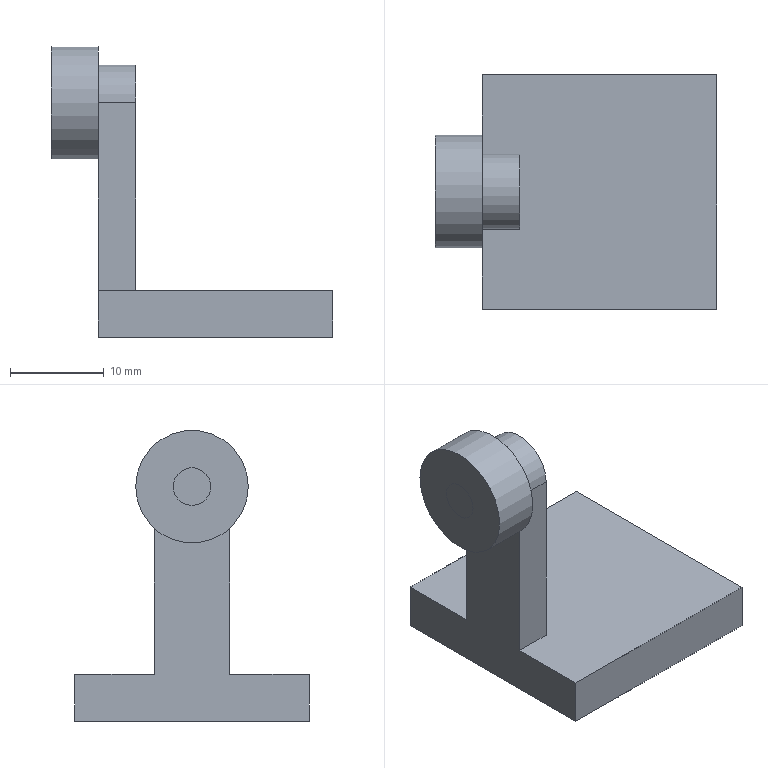Component | NX | FIXED_ROLLER | 2 solids | 16 faces | box 30 x 25 x 31 mm | volume 4431 mm3 | plane 12 | cylinder 4 | commonest cylinder face diameters 4 x2 12 x1 8 x1
STEP:
#1=CARTESIAN_POINT('',(0.,0.,0.));
#2=DIRECTION('',(0.,0.,1.));
#3=DIRECTION('',(1.,0.,0.));
#4=AXIS2_PLACEMENT_3D('',#1,#2,#3);
#5=CARTESIAN_POINT('',(25.,6.,144.));
#6=VERTEX_POINT('',#5);
#7=CARTESIAN_POINT('',(25.,-0.,144.));
#8=DIRECTION('',(1.,0.,0.));
#9=DIRECTION('',(0.,1.,0.));
#10=AXIS2_PLACEMENT_3D('',#7,#8,#9);
#11=CIRCLE('',#10,6.);
#12=CARTESIAN_POINT('',(25.,-0.,144.));
#13=DIRECTION('',(-1.,0.,0.));
#14=DIRECTION('',(0.,0.,1.));
#15=AXIS2_PLACEMENT_3D('',#12,#13,#14);
#16=CYLINDRICAL_SURFACE('',#15,6.);
#17=CARTESIAN_POINT('',(7.854,0.));
#18=DIRECTION('',(-1.,0.));
#19=VECTOR('',#18,1.);
#20=LINE('',#17,#19);
#21=(GEOMETRIC_REPRESENTATION_CONTEXT(2)PARAMETRIC_REPRESENTATION_CONTEXT()REPRESENTATION_CONTEXT('',''));
#22=DEFINITIONAL_REPRESENTATION('',(#20),#21);
#23=PCURVE('',#16,#22);
#24=CARTESIAN_POINT('',(25.,-0.,144.));
#25=DIRECTION('',(1.,0.,0.));
#26=DIRECTION('',(0.,0.,-1.));
#27=AXIS2_PLACEMENT_3D('',#24,#25,#26);
#28=PLANE('',#27);
#29=CARTESIAN_POINT('',(0.,0.));
#30=DIRECTION('',(0.,1.));
#31=AXIS2_PLACEMENT_2D('',#29,#30);
#32=CIRCLE('',#31,6.);
#33=(GEOMETRIC_REPRESENTATION_CONTEXT(2)PARAMETRIC_REPRESENTATION_CONTEXT()REPRESENTATION_CONTEXT('',''));
#34=DEFINITIONAL_REPRESENTATION('',(#32),#33);
#35=PCURVE('',#28,#34);
#36=SURFACE_CURVE('',#11,(#23,#35),.PCURVE_S1.);
#37=EDGE_CURVE('',#6,#6,#36,.T.);
#38=ORIENTED_EDGE('',*,*,#37,.F.);
#39=CARTESIAN_POINT('',(20.,6.,144.));
#40=VERTEX_POINT('',#39);
#41=CARTESIAN_POINT('',(25.,6.,144.));
#42=CARTESIAN_POINT('',(20.,6.,144.));
#43=B_SPLINE_CURVE_WITH_KNOTS('',1,(#41,#42),.UNSPECIFIED.,.F.,.F.,(2,2),(0.,5.),.PIECEWISE_BEZIER_KNOTS.);
#44=CARTESIAN_POINT('',(7.854,0.));
#45=DIRECTION('',(0.,1.));
#46=VECTOR('',#45,1.);
#47=LINE('',#44,#46);
#48=(GEOMETRIC_REPRESENTATION_CONTEXT(2)PARAMETRIC_REPRESENTATION_CONTEXT()REPRESENTATION_CONTEXT('',''));
#49=DEFINITIONAL_REPRESENTATION('',(#47),#48);
#50=PCURVE('',#16,#49);
#51=CARTESIAN_POINT('',(1.571,0.));
#52=DIRECTION('',(0.,1.));
#53=VECTOR('',#52,1.);
#54=LINE('',#51,#53);
#55=(GEOMETRIC_REPRESENTATION_CONTEXT(2)PARAMETRIC_REPRESENTATION_CONTEXT()REPRESENTATION_CONTEXT('',''));
#56=DEFINITIONAL_REPRESENTATION('',(#54),#55);
#57=PCURVE('',#16,#56);
#58=SEAM_CURVE('',#43,(#50,#57),.PCURVE_S1.);
#59=EDGE_CURVE('',#6,#40,#58,.T.);
#60=ORIENTED_EDGE('',*,*,#59,.T.);
#61=CARTESIAN_POINT('',(20.,-0.,144.));
#62=DIRECTION('',(1.,0.,0.));
#63=DIRECTION('',(0.,1.,0.));
#64=AXIS2_PLACEMENT_3D('',#61,#62,#63);
#65=CIRCLE('',#64,6.);
#66=CARTESIAN_POINT('',(7.854,5.));
#67=DIRECTION('',(-1.,0.));
#68=VECTOR('',#67,1.);
#69=LINE('',#66,#68);
#70=(GEOMETRIC_REPRESENTATION_CONTEXT(2)PARAMETRIC_REPRESENTATION_CONTEXT()REPRESENTATION_CONTEXT('',''));
#71=DEFINITIONAL_REPRESENTATION('',(#69),#70);
#72=PCURVE('',#16,#71);
#73=CARTESIAN_POINT('',(20.,-0.,144.));
#74=DIRECTION('',(1.,0.,0.));
#75=DIRECTION('',(0.,0.,-1.));
#76=AXIS2_PLACEMENT_3D('',#73,#74,#75);
#77=PLANE('',#76);
#78=CARTESIAN_POINT('',(0.,0.));
#79=DIRECTION('',(0.,1.));
#80=AXIS2_PLACEMENT_2D('',#78,#79);
#81=CIRCLE('',#80,6.);
#82=(GEOMETRIC_REPRESENTATION_CONTEXT(2)PARAMETRIC_REPRESENTATION_CONTEXT()REPRESENTATION_CONTEXT('',''));
#83=DEFINITIONAL_REPRESENTATION('',(#81),#82);
#84=PCURVE('',#77,#83);
#85=SURFACE_CURVE('',#65,(#72,#84),.PCURVE_S1.);
#86=EDGE_CURVE('',#40,#40,#85,.T.);
#87=ORIENTED_EDGE('',*,*,#86,.T.);
#88=ORIENTED_EDGE('',*,*,#59,.F.);
#89=EDGE_LOOP('',(#38,#60,#87,#88));
#90=FACE_BOUND('',#89,.T.);
#91=ADVANCED_FACE('',(#90),#16,.T.);
#92=CARTESIAN_POINT('',(25.,2.,144.));
#93=VERTEX_POINT('',#92);
#94=CARTESIAN_POINT('',(25.,-0.,144.));
#95=DIRECTION('',(1.,0.,0.));
#96=DIRECTION('',(0.,1.,0.));
#97=AXIS2_PLACEMENT_3D('',#94,#95,#96);
#98=CIRCLE('',#97,2.);
#99=CARTESIAN_POINT('',(25.,-0.,144.));
#100=DIRECTION('',(-1.,0.,0.));
#101=DIRECTION('',(0.,0.,1.));
#102=AXIS2_PLACEMENT_3D('',#99,#100,#101);
#103=CYLINDRICAL_SURFACE('',#102,2.);
#104=CARTESIAN_POINT('',(7.854,0.));
#105=DIRECTION('',(-1.,0.));
#106=VECTOR('',#105,1.);
#107=LINE('',#104,#106);
#108=(GEOMETRIC_REPRESENTATION_CONTEXT(2)PARAMETRIC_REPRESENTATION_CONTEXT()REPRESENTATION_CONTEXT('',''));
#109=DEFINITIONAL_REPRESENTATION('',(#107),#108);
#110=PCURVE('',#103,#109);
#111=CARTESIAN_POINT('',(0.,0.));
#112=DIRECTION('',(0.,1.));
#113=AXIS2_PLACEMENT_2D('',#111,#112);
#114=CIRCLE('',#113,2.);
#115=(GEOMETRIC_REPRESENTATION_CONTEXT(2)PARAMETRIC_REPRESENTATION_CONTEXT()REPRESENTATION_CONTEXT('',''));
#116=DEFINITIONAL_REPRESENTATION('',(#114),#115);
#117=PCURVE('',#28,#116);
#118=SURFACE_CURVE('',#98,(#110,#117),.PCURVE_S1.);
#119=EDGE_CURVE('',#93,#93,#118,.T.);
#120=ORIENTED_EDGE('',*,*,#119,.F.);
#121=CARTESIAN_POINT('',(20.,2.,144.));
#122=VERTEX_POINT('',#121);
#123=CARTESIAN_POINT('',(25.,2.,144.));
#124=CARTESIAN_POINT('',(20.,2.,144.));
#125=B_SPLINE_CURVE_WITH_KNOTS('',1,(#123,#124),.UNSPECIFIED.,.F.,.F.,(2,2),(0.,5.),.PIECEWISE_BEZIER_KNOTS.);
#126=CARTESIAN_POINT('',(7.854,0.));
#127=DIRECTION('',(0.,1.));
#128=VECTOR('',#127,1.);
#129=LINE('',#126,#128);
#130=(GEOMETRIC_REPRESENTATION_CONTEXT(2)PARAMETRIC_REPRESENTATION_CONTEXT()REPRESENTATION_CONTEXT('',''));
#131=DEFINITIONAL_REPRESENTATION('',(#129),#130);
#132=PCURVE('',#103,#131);
#133=CARTESIAN_POINT('',(1.571,0.));
#134=DIRECTION('',(0.,1.));
#135=VECTOR('',#134,1.);
#136=LINE('',#133,#135);
#137=(GEOMETRIC_REPRESENTATION_CONTEXT(2)PARAMETRIC_REPRESENTATION_CONTEXT()REPRESENTATION_CONTEXT('',''));
#138=DEFINITIONAL_REPRESENTATION('',(#136),#137);
#139=PCURVE('',#103,#138);
#140=SEAM_CURVE('',#125,(#132,#139),.PCURVE_S1.);
#141=EDGE_CURVE('',#93,#122,#140,.T.);
#142=ORIENTED_EDGE('',*,*,#141,.T.);
#143=CARTESIAN_POINT('',(20.,-0.,144.));
#144=DIRECTION('',(1.,0.,0.));
#145=DIRECTION('',(0.,1.,0.));
#146=AXIS2_PLACEMENT_3D('',#143,#144,#145);
#147=CIRCLE('',#146,2.);
#148=CARTESIAN_POINT('',(7.854,5.));
#149=DIRECTION('',(-1.,0.));
#150=VECTOR('',#149,1.);
#151=LINE('',#148,#150);
#152=(GEOMETRIC_REPRESENTATION_CONTEXT(2)PARAMETRIC_REPRESENTATION_CONTEXT()REPRESENTATION_CONTEXT('',''));
#153=DEFINITIONAL_REPRESENTATION('',(#151),#152);
#154=PCURVE('',#103,#153);
#155=CARTESIAN_POINT('',(0.,0.));
#156=DIRECTION('',(0.,1.));
#157=AXIS2_PLACEMENT_2D('',#155,#156);
#158=CIRCLE('',#157,2.);
#159=(GEOMETRIC_REPRESENTATION_CONTEXT(2)PARAMETRIC_REPRESENTATION_CONTEXT()REPRESENTATION_CONTEXT('',''));
#160=DEFINITIONAL_REPRESENTATION('',(#158),#159);
#161=PCURVE('',#77,#160);
#162=SURFACE_CURVE('',#147,(#154,#161),.PCURVE_S1.);
#163=EDGE_CURVE('',#122,#122,#162,.T.);
#164=ORIENTED_EDGE('',*,*,#163,.T.);
#165=ORIENTED_EDGE('',*,*,#141,.F.);
#166=EDGE_LOOP('',(#120,#142,#164,#165));
#167=FACE_BOUND('',#166,.F.);
#168=ADVANCED_FACE('',(#167),#103,.F.);
#169=ORIENTED_EDGE('',*,*,#37,.T.);
#170=EDGE_LOOP('',(#169));
#171=FACE_BOUND('',#170,.T.);
#172=ORIENTED_EDGE('',*,*,#119,.F.);
#173=EDGE_LOOP('',(#172));
#174=FACE_BOUND('',#173,.T.);
#175=ADVANCED_FACE('',(#171,#174),#28,.T.);
#176=ORIENTED_EDGE('',*,*,#86,.F.);
#177=EDGE_LOOP('',(#176));
#178=FACE_BOUND('',#177,.T.);
#179=ORIENTED_EDGE('',*,*,#163,.T.);
#180=EDGE_LOOP('',(#179));
#181=FACE_BOUND('',#180,.T.);
#182=ADVANCED_FACE('',(#178,#181),#77,.F.);
#183=CLOSED_SHELL('',(#91,#168,#175,#182));
#184=MANIFOLD_SOLID_BREP('',#183);
#185=(LENGTH_UNIT()NAMED_UNIT(*)SI_UNIT(.MILLI.,.METRE.));
#186=UNCERTAINTY_MEASURE_WITH_UNIT(LENGTH_MEASURE(0.00001),#185,'','');
#187=(NAMED_UNIT(*)PLANE_ANGLE_UNIT()SI_UNIT($,.RADIAN.));
#188=(NAMED_UNIT(*)SI_UNIT($,.STERADIAN.)SOLID_ANGLE_UNIT());
#189=(GEOMETRIC_REPRESENTATION_CONTEXT(3)GLOBAL_UNCERTAINTY_ASSIGNED_CONTEXT((#186))GLOBAL_UNIT_ASSIGNED_CONTEXT((#185,#187,#188))REPRESENTATION_CONTEXT('',''));
#190=ADVANCED_BREP_SHAPE_REPRESENTATION('',(#4,#184),#189);
#191=CARTESIAN_POINT('',(0.,0.,0.));
#192=DIRECTION('',(0.,0.,1.));
#193=DIRECTION('',(1.,0.,0.));
#194=AXIS2_PLACEMENT_3D('',#191,#192,#193);
#195=CARTESIAN_POINT('',(0.,0.,0.));
#196=DIRECTION('',(0.,0.,1.));
#197=DIRECTION('',(1.,0.,0.));
#198=AXIS2_PLACEMENT_3D('',#195,#196,#197);
#199=(LENGTH_UNIT()NAMED_UNIT(*)SI_UNIT(.MILLI.,.METRE.));
#200=UNCERTAINTY_MEASURE_WITH_UNIT(LENGTH_MEASURE(0.000002),#199,'','');
#201=(NAMED_UNIT(*)PLANE_ANGLE_UNIT()SI_UNIT($,.RADIAN.));
#202=(NAMED_UNIT(*)SI_UNIT($,.STERADIAN.)SOLID_ANGLE_UNIT());
#203=(GEOMETRIC_REPRESENTATION_CONTEXT(3)GLOBAL_UNCERTAINTY_ASSIGNED_CONTEXT((#200))GLOBAL_UNIT_ASSIGNED_CONTEXT((#199,#201,#202))REPRESENTATION_CONTEXT('',''));
#204=SHAPE_REPRESENTATION('',(#4,#194,#198),#203);
#205=ITEM_DEFINED_TRANSFORMATION('','',#4,#194);
#206=(REPRESENTATION_RELATIONSHIP('','',#190,#204)REPRESENTATION_RELATIONSHIP_WITH_TRANSFORMATION(#205)SHAPE_REPRESENTATION_RELATIONSHIP());
#207=CARTESIAN_POINT('',(20.,2.,144.));
#208=VERTEX_POINT('',#207);
#209=CARTESIAN_POINT('',(20.,-0.,144.));
#210=DIRECTION('',(-1.,0.,0.));
#211=DIRECTION('',(0.,1.,0.));
#212=AXIS2_PLACEMENT_3D('',#209,#210,#211);
#213=CIRCLE('',#212,2.);
#214=CARTESIAN_POINT('',(20.,-0.,144.));
#215=DIRECTION('',(1.,0.,0.));
#216=DIRECTION('',(0.,0.,-1.));
#217=AXIS2_PLACEMENT_3D('',#214,#215,#216);
#218=CYLINDRICAL_SURFACE('',#217,2.);
#219=CARTESIAN_POINT('',(7.854,0.));
#220=DIRECTION('',(-1.,0.));
#221=VECTOR('',#220,1.);
#222=LINE('',#219,#221);
#223=(GEOMETRIC_REPRESENTATION_CONTEXT(2)PARAMETRIC_REPRESENTATION_CONTEXT()REPRESENTATION_CONTEXT('',''));
#224=DEFINITIONAL_REPRESENTATION('',(#222),#223);
#225=PCURVE('',#218,#224);
#226=CARTESIAN_POINT('',(20.,-0.,144.));
#227=DIRECTION('',(-1.,0.,0.));
#228=DIRECTION('',(0.,0.,1.));
#229=AXIS2_PLACEMENT_3D('',#226,#227,#228);
#230=PLANE('',#229);
#231=CARTESIAN_POINT('',(0.,0.));
#232=DIRECTION('',(0.,1.));
#233=AXIS2_PLACEMENT_2D('',#231,#232);
#234=CIRCLE('',#233,2.);
#235=(GEOMETRIC_REPRESENTATION_CONTEXT(2)PARAMETRIC_REPRESENTATION_CONTEXT()REPRESENTATION_CONTEXT('',''));
#236=DEFINITIONAL_REPRESENTATION('',(#234),#235);
#237=PCURVE('',#230,#236);
#238=SURFACE_CURVE('',#213,(#225,#237),.PCURVE_S1.);
#239=EDGE_CURVE('',#208,#208,#238,.T.);
#240=ORIENTED_EDGE('',*,*,#239,.F.);
#241=CARTESIAN_POINT('',(25.,2.,144.));
#242=VERTEX_POINT('',#241);
#243=CARTESIAN_POINT('',(20.,2.,144.));
#244=CARTESIAN_POINT('',(25.,2.,144.));
#245=B_SPLINE_CURVE_WITH_KNOTS('',1,(#243,#244),.UNSPECIFIED.,.F.,.F.,(2,2),(0.,5.),.PIECEWISE_BEZIER_KNOTS.);
#246=CARTESIAN_POINT('',(7.854,0.));
#247=DIRECTION('',(0.,1.));
#248=VECTOR('',#247,1.);
#249=LINE('',#246,#248);
#250=(GEOMETRIC_REPRESENTATION_CONTEXT(2)PARAMETRIC_REPRESENTATION_CONTEXT()REPRESENTATION_CONTEXT('',''));
#251=DEFINITIONAL_REPRESENTATION('',(#249),#250);
#252=PCURVE('',#218,#251);
#253=CARTESIAN_POINT('',(1.571,0.));
#254=DIRECTION('',(0.,1.));
#255=VECTOR('',#254,1.);
#256=LINE('',#253,#255);
#257=(GEOMETRIC_REPRESENTATION_CONTEXT(2)PARAMETRIC_REPRESENTATION_CONTEXT()REPRESENTATION_CONTEXT('',''));
#258=DEFINITIONAL_REPRESENTATION('',(#256),#257);
#259=PCURVE('',#218,#258);
#260=SEAM_CURVE('',#245,(#252,#259),.PCURVE_S1.);
#261=EDGE_CURVE('',#208,#242,#260,.T.);
#262=ORIENTED_EDGE('',*,*,#261,.T.);
#263=CARTESIAN_POINT('',(25.,-0.,144.));
#264=DIRECTION('',(-1.,0.,0.));
#265=DIRECTION('',(0.,1.,0.));
#266=AXIS2_PLACEMENT_3D('',#263,#264,#265);
#267=CIRCLE('',#266,2.);
#268=CARTESIAN_POINT('',(7.854,5.));
#269=DIRECTION('',(-1.,0.));
#270=VECTOR('',#269,1.);
#271=LINE('',#268,#270);
#272=(GEOMETRIC_REPRESENTATION_CONTEXT(2)PARAMETRIC_REPRESENTATION_CONTEXT()REPRESENTATION_CONTEXT('',''));
#273=DEFINITIONAL_REPRESENTATION('',(#271),#272);
#274=PCURVE('',#218,#273);
#275=CARTESIAN_POINT('',(25.,-0.,144.));
#276=DIRECTION('',(1.,0.,0.));
#277=DIRECTION('',(0.,0.,-1.));
#278=AXIS2_PLACEMENT_3D('',#275,#276,#277);
#279=PLANE('',#278);
#280=CARTESIAN_POINT('',(0.,2.));
#281=CARTESIAN_POINT('',(3.464,2.));
#282=CARTESIAN_POINT('',(1.732,-1.));
#283=CARTESIAN_POINT('',(0.,-4.));
#284=CARTESIAN_POINT('',(-1.732,-1.));
#285=CARTESIAN_POINT('',(-3.464,2.));
#286=CARTESIAN_POINT('',(0.,2.));
#287=(BOUNDED_CURVE()B_SPLINE_CURVE(2,(#280,#281,#282,#283,#284,#285,#286),.UNSPECIFIED.,.T.,.F.)B_SPLINE_CURVE_WITH_KNOTS((1,2,2,2,2,1),(-2.094,0.,2.094,4.189,6.283,8.378),.UNSPECIFIED.)CURVE()GEOMETRIC_REPRESENTATION_ITEM()RATIONAL_B_SPLINE_CURVE((1.,0.5,1.,0.5,1.,0.5,1.))REPRESENTATION_ITEM(''));
#288=(GEOMETRIC_REPRESENTATION_CONTEXT(2)PARAMETRIC_REPRESENTATION_CONTEXT()REPRESENTATION_CONTEXT('',''));
#289=DEFINITIONAL_REPRESENTATION('',(#287),#288);
#290=PCURVE('',#279,#289);
#291=SURFACE_CURVE('',#267,(#274,#290),.PCURVE_S1.);
#292=EDGE_CURVE('',#242,#242,#291,.T.);
#293=ORIENTED_EDGE('',*,*,#292,.T.);
#294=ORIENTED_EDGE('',*,*,#261,.F.);
#295=EDGE_LOOP('',(#240,#262,#293,#294));
#296=FACE_BOUND('',#295,.T.);
#297=ADVANCED_FACE('',(#296),#218,.T.);
#298=ORIENTED_EDGE('',*,*,#239,.T.);
#299=EDGE_LOOP('',(#298));
#300=FACE_BOUND('',#299,.T.);
#301=ADVANCED_FACE('',(#300),#230,.T.);
#302=CARTESIAN_POINT('',(25.,-4.,144.));
#303=VERTEX_POINT('',#302);
#304=CARTESIAN_POINT('',(25.,-4.,124.));
#305=VERTEX_POINT('',#304);
#306=CARTESIAN_POINT('',(25.,-4.,144.));
#307=DIRECTION('',(0.,0.,-1.));
#308=VECTOR('',#307,1.);
#309=LINE('',#306,#308);
#310=CARTESIAN_POINT('',(29.,-4.,144.));
#311=DIRECTION('',(0.,1.,0.));
#312=DIRECTION('',(0.,-0.,1.));
#313=AXIS2_PLACEMENT_3D('',#310,#311,#312);
#314=PLANE('',#313);
#315=CARTESIAN_POINT('',(0.,-4.));
#316=DIRECTION('',(-1.,0.));
#317=VECTOR('',#316,1.);
#318=LINE('',#315,#317);
#319=(GEOMETRIC_REPRESENTATION_CONTEXT(2)PARAMETRIC_REPRESENTATION_CONTEXT()REPRESENTATION_CONTEXT('',''));
#320=DEFINITIONAL_REPRESENTATION('',(#318),#319);
#321=PCURVE('',#314,#320);
#322=CARTESIAN_POINT('',(0.,-4.));
#323=DIRECTION('',(1.,0.));
#324=VECTOR('',#323,1.);
#325=LINE('',#322,#324);
#326=(GEOMETRIC_REPRESENTATION_CONTEXT(2)PARAMETRIC_REPRESENTATION_CONTEXT()REPRESENTATION_CONTEXT('',''));
#327=DEFINITIONAL_REPRESENTATION('',(#325),#326);
#328=PCURVE('',#279,#327);
#329=SURFACE_CURVE('',#309,(#321,#328),.PCURVE_S1.);
#330=EDGE_CURVE('',#303,#305,#329,.T.);
#331=ORIENTED_EDGE('',*,*,#330,.T.);
#332=CARTESIAN_POINT('',(29.,-4.,124.));
#333=VERTEX_POINT('',#332);
#334=CARTESIAN_POINT('',(29.,-4.,124.));
#335=DIRECTION('',(-1.,0.,0.));
#336=VECTOR('',#335,1.);
#337=LINE('',#334,#336);
#338=CARTESIAN_POINT('',(-20.,0.));
#339=DIRECTION('',(0.,-1.));
#340=VECTOR('',#339,1.);
#341=LINE('',#338,#340);
#342=(GEOMETRIC_REPRESENTATION_CONTEXT(2)PARAMETRIC_REPRESENTATION_CONTEXT()REPRESENTATION_CONTEXT('',''));
#343=DEFINITIONAL_REPRESENTATION('',(#341),#342);
#344=PCURVE('',#314,#343);
#345=CARTESIAN_POINT('',(50.,-12.5,124.));
#346=DIRECTION('',(0.,0.,1.));
#347=DIRECTION('',(0.,-1.,0.));
#348=AXIS2_PLACEMENT_3D('',#345,#346,#347);
#349=PLANE('',#348);
#350=CARTESIAN_POINT('',(-8.5,-21.));
#351=DIRECTION('',(0.,-1.));
#352=VECTOR('',#351,1.);
#353=LINE('',#350,#352);
#354=(GEOMETRIC_REPRESENTATION_CONTEXT(2)PARAMETRIC_REPRESENTATION_CONTEXT()REPRESENTATION_CONTEXT('',''));
#355=DEFINITIONAL_REPRESENTATION('',(#353),#354);
#356=PCURVE('',#349,#355);
#357=SURFACE_CURVE('',#337,(#344,#356),.PCURVE_S1.);
#358=EDGE_CURVE('',#333,#305,#357,.T.);
#359=ORIENTED_EDGE('',*,*,#358,.F.);
#360=CARTESIAN_POINT('',(29.,-4.,144.));
#361=VERTEX_POINT('',#360);
#362=CARTESIAN_POINT('',(29.,-4.,144.));
#363=DIRECTION('',(0.,0.,-1.));
#364=VECTOR('',#363,1.);
#365=LINE('',#362,#364);
#366=CARTESIAN_POINT('',(0.,0.));
#367=DIRECTION('',(-1.,0.));
#368=VECTOR('',#367,1.);
#369=LINE('',#366,#368);
#370=(GEOMETRIC_REPRESENTATION_CONTEXT(2)PARAMETRIC_REPRESENTATION_CONTEXT()REPRESENTATION_CONTEXT('',''));
#371=DEFINITIONAL_REPRESENTATION('',(#369),#370);
#372=PCURVE('',#314,#371);
#373=CARTESIAN_POINT('',(29.,-0.,144.));
#374=DIRECTION('',(1.,0.,0.));
#375=DIRECTION('',(0.,0.,-1.));
#376=AXIS2_PLACEMENT_3D('',#373,#374,#375);
#377=PLANE('',#376);
#378=CARTESIAN_POINT('',(0.,-4.));
#379=DIRECTION('',(1.,0.));
#380=VECTOR('',#379,1.);
#381=LINE('',#378,#380);
#382=(GEOMETRIC_REPRESENTATION_CONTEXT(2)PARAMETRIC_REPRESENTATION_CONTEXT()REPRESENTATION_CONTEXT('',''));
#383=DEFINITIONAL_REPRESENTATION('',(#381),#382);
#384=PCURVE('',#377,#383);
#385=SURFACE_CURVE('',#365,(#372,#384),.PCURVE_S1.);
#386=EDGE_CURVE('',#361,#333,#385,.T.);
#387=ORIENTED_EDGE('',*,*,#386,.F.);
#388=CARTESIAN_POINT('',(29.,-4.,144.));
#389=DIRECTION('',(-1.,0.,0.));
#390=VECTOR('',#389,1.);
#391=LINE('',#388,#390);
#392=CARTESIAN_POINT('',(0.,0.));
#393=DIRECTION('',(0.,-1.));
#394=VECTOR('',#393,1.);
#395=LINE('',#392,#394);
#396=(GEOMETRIC_REPRESENTATION_CONTEXT(2)PARAMETRIC_REPRESENTATION_CONTEXT()REPRESENTATION_CONTEXT('',''));
#397=DEFINITIONAL_REPRESENTATION('',(#395),#396);
#398=PCURVE('',#314,#397);
#399=CARTESIAN_POINT('',(29.,-0.,144.));
#400=DIRECTION('',(-1.,0.,0.));
#401=DIRECTION('',(0.,0.,1.));
#402=AXIS2_PLACEMENT_3D('',#399,#400,#401);
#403=CYLINDRICAL_SURFACE('',#402,4.);
#404=CARTESIAN_POINT('',(-1.571,0.));
#405=DIRECTION('',(0.,1.));
#406=VECTOR('',#405,1.);
#407=LINE('',#404,#406);
#408=(GEOMETRIC_REPRESENTATION_CONTEXT(2)PARAMETRIC_REPRESENTATION_CONTEXT()REPRESENTATION_CONTEXT('',''));
#409=DEFINITIONAL_REPRESENTATION('',(#407),#408);
#410=PCURVE('',#403,#409);
#411=SURFACE_CURVE('',#391,(#398,#410),.PCURVE_S1.);
#412=EDGE_CURVE('',#361,#303,#411,.T.);
#413=ORIENTED_EDGE('',*,*,#412,.T.);
#414=EDGE_LOOP('',(#331,#359,#387,#413));
#415=FACE_BOUND('',#414,.T.);
#416=ADVANCED_FACE('',(#415),#314,.F.);
#417=CARTESIAN_POINT('',(25.,4.,124.));
#418=VERTEX_POINT('',#417);
#419=CARTESIAN_POINT('',(25.,4.,144.));
#420=VERTEX_POINT('',#419);
#421=CARTESIAN_POINT('',(25.,4.,124.));
#422=DIRECTION('',(0.,-0.,1.));
#423=VECTOR('',#422,1.);
#424=LINE('',#421,#423);
#425=CARTESIAN_POINT('',(29.,4.,124.));
#426=DIRECTION('',(0.,-1.,-0.));
#427=DIRECTION('',(0.,0.,-1.));
#428=AXIS2_PLACEMENT_3D('',#425,#426,#427);
#429=PLANE('',#428);
#430=CARTESIAN_POINT('',(0.,-4.));
#431=DIRECTION('',(-1.,0.));
#432=VECTOR('',#431,1.);
#433=LINE('',#430,#432);
#434=(GEOMETRIC_REPRESENTATION_CONTEXT(2)PARAMETRIC_REPRESENTATION_CONTEXT()REPRESENTATION_CONTEXT('',''));
#435=DEFINITIONAL_REPRESENTATION('',(#433),#434);
#436=PCURVE('',#429,#435);
#437=CARTESIAN_POINT('',(20.,4.));
#438=DIRECTION('',(-1.,-0.));
#439=VECTOR('',#438,1.);
#440=LINE('',#437,#439);
#441=(GEOMETRIC_REPRESENTATION_CONTEXT(2)PARAMETRIC_REPRESENTATION_CONTEXT()REPRESENTATION_CONTEXT('',''));
#442=DEFINITIONAL_REPRESENTATION('',(#440),#441);
#443=PCURVE('',#279,#442);
#444=SURFACE_CURVE('',#424,(#436,#443),.PCURVE_S1.);
#445=EDGE_CURVE('',#418,#420,#444,.T.);
#446=ORIENTED_EDGE('',*,*,#445,.T.);
#447=CARTESIAN_POINT('',(29.,4.,144.));
#448=VERTEX_POINT('',#447);
#449=CARTESIAN_POINT('',(29.,4.,144.));
#450=DIRECTION('',(-1.,0.,0.));
#451=VECTOR('',#450,1.);
#452=LINE('',#449,#451);
#453=CARTESIAN_POINT('',(-20.,0.));
#454=DIRECTION('',(0.,-1.));
#455=VECTOR('',#454,1.);
#456=LINE('',#453,#455);
#457=(GEOMETRIC_REPRESENTATION_CONTEXT(2)PARAMETRIC_REPRESENTATION_CONTEXT()REPRESENTATION_CONTEXT('',''));
#458=DEFINITIONAL_REPRESENTATION('',(#456),#457);
#459=PCURVE('',#429,#458);
#460=CARTESIAN_POINT('',(1.571,0.));
#461=DIRECTION('',(0.,1.));
#462=VECTOR('',#461,1.);
#463=LINE('',#460,#462);
#464=(GEOMETRIC_REPRESENTATION_CONTEXT(2)PARAMETRIC_REPRESENTATION_CONTEXT()REPRESENTATION_CONTEXT('',''));
#465=DEFINITIONAL_REPRESENTATION('',(#463),#464);
#466=PCURVE('',#403,#465);
#467=SURFACE_CURVE('',#452,(#459,#466),.PCURVE_S1.);
#468=EDGE_CURVE('',#448,#420,#467,.T.);
#469=ORIENTED_EDGE('',*,*,#468,.F.);
#470=CARTESIAN_POINT('',(29.,4.,124.));
#471=VERTEX_POINT('',#470);
#472=CARTESIAN_POINT('',(29.,4.,124.));
#473=DIRECTION('',(0.,-0.,1.));
#474=VECTOR('',#473,1.);
#475=LINE('',#472,#474);
#476=CARTESIAN_POINT('',(0.,0.));
#477=DIRECTION('',(-1.,0.));
#478=VECTOR('',#477,1.);
#479=LINE('',#476,#478);
#480=(GEOMETRIC_REPRESENTATION_CONTEXT(2)PARAMETRIC_REPRESENTATION_CONTEXT()REPRESENTATION_CONTEXT('',''));
#481=DEFINITIONAL_REPRESENTATION('',(#479),#480);
#482=PCURVE('',#429,#481);
#483=CARTESIAN_POINT('',(20.,4.));
#484=DIRECTION('',(-1.,-0.));
#485=VECTOR('',#484,1.);
#486=LINE('',#483,#485);
#487=(GEOMETRIC_REPRESENTATION_CONTEXT(2)PARAMETRIC_REPRESENTATION_CONTEXT()REPRESENTATION_CONTEXT('',''));
#488=DEFINITIONAL_REPRESENTATION('',(#486),#487);
#489=PCURVE('',#377,#488);
#490=SURFACE_CURVE('',#475,(#482,#489),.PCURVE_S1.);
#491=EDGE_CURVE('',#471,#448,#490,.T.);
#492=ORIENTED_EDGE('',*,*,#491,.F.);
#493=CARTESIAN_POINT('',(29.,4.,124.));
#494=DIRECTION('',(-1.,0.,0.));
#495=VECTOR('',#494,1.);
#496=LINE('',#493,#495);
#497=CARTESIAN_POINT('',(0.,0.));
#498=DIRECTION('',(0.,-1.));
#499=VECTOR('',#498,1.);
#500=LINE('',#497,#499);
#501=(GEOMETRIC_REPRESENTATION_CONTEXT(2)PARAMETRIC_REPRESENTATION_CONTEXT()REPRESENTATION_CONTEXT('',''));
#502=DEFINITIONAL_REPRESENTATION('',(#500),#501);
#503=PCURVE('',#429,#502);
#504=CARTESIAN_POINT('',(-16.5,-21.));
#505=DIRECTION('',(0.,-1.));
#506=VECTOR('',#505,1.);
#507=LINE('',#504,#506);
#508=(GEOMETRIC_REPRESENTATION_CONTEXT(2)PARAMETRIC_REPRESENTATION_CONTEXT()REPRESENTATION_CONTEXT('',''));
#509=DEFINITIONAL_REPRESENTATION('',(#507),#508);
#510=PCURVE('',#349,#509);
#511=SURFACE_CURVE('',#496,(#503,#510),.PCURVE_S1.);
#512=EDGE_CURVE('',#471,#418,#511,.T.);
#513=ORIENTED_EDGE('',*,*,#512,.T.);
#514=EDGE_LOOP('',(#446,#469,#492,#513));
#515=FACE_BOUND('',#514,.T.);
#516=ADVANCED_FACE('',(#515),#429,.F.);
#517=CARTESIAN_POINT('',(25.,-0.,144.));
#518=DIRECTION('',(1.,0.,0.));
#519=DIRECTION('',(0.,1.,0.));
#520=AXIS2_PLACEMENT_3D('',#517,#518,#519);
#521=CIRCLE('',#520,4.);
#522=CARTESIAN_POINT('',(1.571,4.));
#523=DIRECTION('',(-1.,0.));
#524=VECTOR('',#523,1.);
#525=LINE('',#522,#524);
#526=(GEOMETRIC_REPRESENTATION_CONTEXT(2)PARAMETRIC_REPRESENTATION_CONTEXT()REPRESENTATION_CONTEXT('',''));
#527=DEFINITIONAL_REPRESENTATION('',(#525),#526);
#528=PCURVE('',#403,#527);
#529=CARTESIAN_POINT('',(0.,0.));
#530=DIRECTION('',(0.,1.));
#531=AXIS2_PLACEMENT_2D('',#529,#530);
#532=CIRCLE('',#531,4.);
#533=(GEOMETRIC_REPRESENTATION_CONTEXT(2)PARAMETRIC_REPRESENTATION_CONTEXT()REPRESENTATION_CONTEXT('',''));
#534=DEFINITIONAL_REPRESENTATION('',(#532),#533);
#535=PCURVE('',#279,#534);
#536=SURFACE_CURVE('',#521,(#528,#535),.PCURVE_S1.);
#537=EDGE_CURVE('',#420,#303,#536,.T.);
#538=ORIENTED_EDGE('',*,*,#537,.T.);
#539=ORIENTED_EDGE('',*,*,#412,.F.);
#540=CARTESIAN_POINT('',(29.,-0.,144.));
#541=DIRECTION('',(1.,0.,0.));
#542=DIRECTION('',(0.,1.,0.));
#543=AXIS2_PLACEMENT_3D('',#540,#541,#542);
#544=CIRCLE('',#543,4.);
#545=CARTESIAN_POINT('',(1.571,0.));
#546=DIRECTION('',(-1.,0.));
#547=VECTOR('',#546,1.);
#548=LINE('',#545,#547);
#549=(GEOMETRIC_REPRESENTATION_CONTEXT(2)PARAMETRIC_REPRESENTATION_CONTEXT()REPRESENTATION_CONTEXT('',''));
#550=DEFINITIONAL_REPRESENTATION('',(#548),#549);
#551=PCURVE('',#403,#550);
#552=CARTESIAN_POINT('',(0.,0.));
#553=DIRECTION('',(0.,1.));
#554=AXIS2_PLACEMENT_2D('',#552,#553);
#555=CIRCLE('',#554,4.);
#556=(GEOMETRIC_REPRESENTATION_CONTEXT(2)PARAMETRIC_REPRESENTATION_CONTEXT()REPRESENTATION_CONTEXT('',''));
#557=DEFINITIONAL_REPRESENTATION('',(#555),#556);
#558=PCURVE('',#377,#557);
#559=SURFACE_CURVE('',#544,(#551,#558),.PCURVE_S1.);
#560=EDGE_CURVE('',#448,#361,#559,.T.);
#561=ORIENTED_EDGE('',*,*,#560,.F.);
#562=ORIENTED_EDGE('',*,*,#468,.T.);
#563=EDGE_LOOP('',(#538,#539,#561,#562));
#564=FACE_BOUND('',#563,.T.);
#565=ADVANCED_FACE('',(#564),#403,.T.);
#566=ORIENTED_EDGE('',*,*,#386,.T.);
#567=CARTESIAN_POINT('',(29.,-4.,124.));
#568=DIRECTION('',(0.,1.,0.));
#569=VECTOR('',#568,1.);
#570=LINE('',#567,#569);
#571=CARTESIAN_POINT('',(20.,-4.));
#572=DIRECTION('',(0.,1.));
#573=VECTOR('',#572,1.);
#574=LINE('',#571,#573);
#575=(GEOMETRIC_REPRESENTATION_CONTEXT(2)PARAMETRIC_REPRESENTATION_CONTEXT()REPRESENTATION_CONTEXT('',''));
#576=DEFINITIONAL_REPRESENTATION('',(#574),#575);
#577=PCURVE('',#377,#576);
#578=CARTESIAN_POINT('',(-8.5,-21.));
#579=DIRECTION('',(-1.,0.));
#580=VECTOR('',#579,1.);
#581=LINE('',#578,#580);
#582=(GEOMETRIC_REPRESENTATION_CONTEXT(2)PARAMETRIC_REPRESENTATION_CONTEXT()REPRESENTATION_CONTEXT('',''));
#583=DEFINITIONAL_REPRESENTATION('',(#581),#582);
#584=PCURVE('',#349,#583);
#585=SURFACE_CURVE('',#570,(#577,#584),.PCURVE_S1.);
#586=EDGE_CURVE('',#333,#471,#585,.T.);
#587=ORIENTED_EDGE('',*,*,#586,.T.);
#588=ORIENTED_EDGE('',*,*,#491,.T.);
#589=ORIENTED_EDGE('',*,*,#560,.T.);
#590=EDGE_LOOP('',(#566,#587,#588,#589));
#591=FACE_BOUND('',#590,.T.);
#592=ADVANCED_FACE('',(#591),#377,.T.);
#593=ORIENTED_EDGE('',*,*,#292,.F.);
#594=EDGE_LOOP('',(#593));
#595=FACE_BOUND('',#594,.T.);
#596=ORIENTED_EDGE('',*,*,#330,.F.);
#597=ORIENTED_EDGE('',*,*,#537,.F.);
#598=ORIENTED_EDGE('',*,*,#445,.F.);
#599=CARTESIAN_POINT('',(25.,12.5,124.));
#600=VERTEX_POINT('',#599);
#601=CARTESIAN_POINT('',(25.,-12.5,124.));
#602=DIRECTION('',(0.,1.,-0.));
#603=VECTOR('',#602,1.);
#604=LINE('',#601,#603);
#605=CARTESIAN_POINT('',(20.,-12.5));
#606=DIRECTION('',(0.,1.));
#607=VECTOR('',#606,1.);
#608=LINE('',#605,#607);
#609=(GEOMETRIC_REPRESENTATION_CONTEXT(2)PARAMETRIC_REPRESENTATION_CONTEXT()REPRESENTATION_CONTEXT('',''));
#610=DEFINITIONAL_REPRESENTATION('',(#608),#609);
#611=PCURVE('',#279,#610);
#612=CARTESIAN_POINT('',(0.,-25.));
#613=DIRECTION('',(-1.,0.));
#614=VECTOR('',#613,1.);
#615=LINE('',#612,#614);
#616=(GEOMETRIC_REPRESENTATION_CONTEXT(2)PARAMETRIC_REPRESENTATION_CONTEXT()REPRESENTATION_CONTEXT('',''));
#617=DEFINITIONAL_REPRESENTATION('',(#615),#616);
#618=PCURVE('',#349,#617);
#619=SURFACE_CURVE('',#604,(#611,#618),.PCURVE_S1.);
#620=EDGE_CURVE('',#418,#600,#619,.T.);
#621=ORIENTED_EDGE('',*,*,#620,.T.);
#622=CARTESIAN_POINT('',(25.,12.5,119.));
#623=VERTEX_POINT('',#622);
#624=CARTESIAN_POINT('',(25.,12.5,124.));
#625=DIRECTION('',(0.,-0.,-1.));
#626=VECTOR('',#625,1.);
#627=LINE('',#624,#626);
#628=CARTESIAN_POINT('',(20.,12.5));
#629=DIRECTION('',(1.,-0.));
#630=VECTOR('',#629,1.);
#631=LINE('',#628,#630);
#632=(GEOMETRIC_REPRESENTATION_CONTEXT(2)PARAMETRIC_REPRESENTATION_CONTEXT()REPRESENTATION_CONTEXT('',''));
#633=DEFINITIONAL_REPRESENTATION('',(#631),#632);
#634=PCURVE('',#279,#633);
#635=CARTESIAN_POINT('',(50.,12.5,124.));
#636=DIRECTION('',(0.,1.,-0.));
#637=DIRECTION('',(0.,0.,1.));
#638=AXIS2_PLACEMENT_3D('',#635,#636,#637);
#639=PLANE('',#638);
#640=CARTESIAN_POINT('',(0.,-25.));
#641=DIRECTION('',(-1.,0.));
#642=VECTOR('',#641,1.);
#643=LINE('',#640,#642);
#644=(GEOMETRIC_REPRESENTATION_CONTEXT(2)PARAMETRIC_REPRESENTATION_CONTEXT()REPRESENTATION_CONTEXT('',''));
#645=DEFINITIONAL_REPRESENTATION('',(#643),#644);
#646=PCURVE('',#639,#645);
#647=SURFACE_CURVE('',#627,(#634,#646),.PCURVE_S1.);
#648=EDGE_CURVE('',#600,#623,#647,.T.);
#649=ORIENTED_EDGE('',*,*,#648,.T.);
#650=CARTESIAN_POINT('',(25.,-12.5,119.));
#651=VERTEX_POINT('',#650);
#652=CARTESIAN_POINT('',(25.,12.5,119.));
#653=DIRECTION('',(0.,-1.,0.));
#654=VECTOR('',#653,1.);
#655=LINE('',#652,#654);
#656=CARTESIAN_POINT('',(25.,12.5));
#657=DIRECTION('',(-0.,-1.));
#658=VECTOR('',#657,1.);
#659=LINE('',#656,#658);
#660=(GEOMETRIC_REPRESENTATION_CONTEXT(2)PARAMETRIC_REPRESENTATION_CONTEXT()REPRESENTATION_CONTEXT('',''));
#661=DEFINITIONAL_REPRESENTATION('',(#659),#660);
#662=PCURVE('',#279,#661);
#663=CARTESIAN_POINT('',(50.,12.5,119.));
#664=DIRECTION('',(0.,-0.,-1.));
#665=DIRECTION('',(0.,1.,-0.));
#666=AXIS2_PLACEMENT_3D('',#663,#664,#665);
#667=PLANE('',#666);
#668=CARTESIAN_POINT('',(0.,-25.));
#669=DIRECTION('',(-1.,0.));
#670=VECTOR('',#669,1.);
#671=LINE('',#668,#670);
#672=(GEOMETRIC_REPRESENTATION_CONTEXT(2)PARAMETRIC_REPRESENTATION_CONTEXT()REPRESENTATION_CONTEXT('',''));
#673=DEFINITIONAL_REPRESENTATION('',(#671),#672);
#674=PCURVE('',#667,#673);
#675=SURFACE_CURVE('',#655,(#662,#674),.PCURVE_S1.);
#676=EDGE_CURVE('',#623,#651,#675,.T.);
#677=ORIENTED_EDGE('',*,*,#676,.T.);
#678=CARTESIAN_POINT('',(25.,-12.5,124.));
#679=VERTEX_POINT('',#678);
#680=CARTESIAN_POINT('',(25.,-12.5,119.));
#681=DIRECTION('',(0.,0.,1.));
#682=VECTOR('',#681,1.);
#683=LINE('',#680,#682);
#684=CARTESIAN_POINT('',(25.,-12.5));
#685=DIRECTION('',(-1.,0.));
#686=VECTOR('',#685,1.);
#687=LINE('',#684,#686);
#688=(GEOMETRIC_REPRESENTATION_CONTEXT(2)PARAMETRIC_REPRESENTATION_CONTEXT()REPRESENTATION_CONTEXT('',''));
#689=DEFINITIONAL_REPRESENTATION('',(#687),#688);
#690=PCURVE('',#279,#689);
#691=CARTESIAN_POINT('',(50.,-12.5,119.));
#692=DIRECTION('',(0.,-1.,0.));
#693=DIRECTION('',(0.,0.,-1.));
#694=AXIS2_PLACEMENT_3D('',#691,#692,#693);
#695=PLANE('',#694);
#696=CARTESIAN_POINT('',(0.,-25.));
#697=DIRECTION('',(-1.,0.));
#698=VECTOR('',#697,1.);
#699=LINE('',#696,#698);
#700=(GEOMETRIC_REPRESENTATION_CONTEXT(2)PARAMETRIC_REPRESENTATION_CONTEXT()REPRESENTATION_CONTEXT('',''));
#701=DEFINITIONAL_REPRESENTATION('',(#699),#700);
#702=PCURVE('',#695,#701);
#703=SURFACE_CURVE('',#683,(#690,#702),.PCURVE_S1.);
#704=EDGE_CURVE('',#651,#679,#703,.T.);
#705=ORIENTED_EDGE('',*,*,#704,.T.);
#706=CARTESIAN_POINT('',(25.,-12.5,124.));
#707=DIRECTION('',(0.,1.,-0.));
#708=VECTOR('',#707,1.);
#709=LINE('',#706,#708);
#710=CARTESIAN_POINT('',(20.,-12.5));
#711=DIRECTION('',(0.,1.));
#712=VECTOR('',#711,1.);
#713=LINE('',#710,#712);
#714=(GEOMETRIC_REPRESENTATION_CONTEXT(2)PARAMETRIC_REPRESENTATION_CONTEXT()REPRESENTATION_CONTEXT('',''));
#715=DEFINITIONAL_REPRESENTATION('',(#713),#714);
#716=PCURVE('',#279,#715);
#717=CARTESIAN_POINT('',(0.,-25.));
#718=DIRECTION('',(-1.,0.));
#719=VECTOR('',#718,1.);
#720=LINE('',#717,#719);
#721=(GEOMETRIC_REPRESENTATION_CONTEXT(2)PARAMETRIC_REPRESENTATION_CONTEXT()REPRESENTATION_CONTEXT('',''));
#722=DEFINITIONAL_REPRESENTATION('',(#720),#721);
#723=PCURVE('',#349,#722);
#724=SURFACE_CURVE('',#709,(#716,#723),.PCURVE_S1.);
#725=EDGE_CURVE('',#679,#305,#724,.T.);
#726=ORIENTED_EDGE('',*,*,#725,.T.);
#727=EDGE_LOOP('',(#596,#597,#598,#621,#649,#677,#705,#726));
#728=FACE_BOUND('',#727,.T.);
#729=ADVANCED_FACE('',(#595,#728),#279,.F.);
#730=ORIENTED_EDGE('',*,*,#512,.F.);
#731=ORIENTED_EDGE('',*,*,#586,.F.);
#732=ORIENTED_EDGE('',*,*,#358,.T.);
#733=ORIENTED_EDGE('',*,*,#725,.F.);
#734=CARTESIAN_POINT('',(50.,-12.5,124.));
#735=VERTEX_POINT('',#734);
#736=CARTESIAN_POINT('',(50.,-12.5,124.));
#737=DIRECTION('',(-1.,0.,0.));
#738=VECTOR('',#737,1.);
#739=LINE('',#736,#738);
#740=CARTESIAN_POINT('',(0.,0.));
#741=DIRECTION('',(0.,-1.));
#742=VECTOR('',#741,1.);
#743=LINE('',#740,#742);
#744=(GEOMETRIC_REPRESENTATION_CONTEXT(2)PARAMETRIC_REPRESENTATION_CONTEXT()REPRESENTATION_CONTEXT('',''));
#745=DEFINITIONAL_REPRESENTATION('',(#743),#744);
#746=PCURVE('',#349,#745);
#747=CARTESIAN_POINT('',(-5.,0.));
#748=DIRECTION('',(0.,-1.));
#749=VECTOR('',#748,1.);
#750=LINE('',#747,#749);
#751=(GEOMETRIC_REPRESENTATION_CONTEXT(2)PARAMETRIC_REPRESENTATION_CONTEXT()REPRESENTATION_CONTEXT('',''));
#752=DEFINITIONAL_REPRESENTATION('',(#750),#751);
#753=PCURVE('',#695,#752);
#754=SURFACE_CURVE('',#739,(#746,#753),.PCURVE_S1.);
#755=EDGE_CURVE('',#735,#679,#754,.T.);
#756=ORIENTED_EDGE('',*,*,#755,.F.);
#757=CARTESIAN_POINT('',(50.,12.5,124.));
#758=VERTEX_POINT('',#757);
#759=CARTESIAN_POINT('',(50.,-12.5,124.));
#760=DIRECTION('',(0.,1.,-0.));
#761=VECTOR('',#760,1.);
#762=LINE('',#759,#761);
#763=CARTESIAN_POINT('',(0.,0.));
#764=DIRECTION('',(-1.,0.));
#765=VECTOR('',#764,1.);
#766=LINE('',#763,#765);
#767=(GEOMETRIC_REPRESENTATION_CONTEXT(2)PARAMETRIC_REPRESENTATION_CONTEXT()REPRESENTATION_CONTEXT('',''));
#768=DEFINITIONAL_REPRESENTATION('',(#766),#767);
#769=PCURVE('',#349,#768);
#770=CARTESIAN_POINT('',(50.,-0.,144.));
#771=DIRECTION('',(-1.,0.,0.));
#772=DIRECTION('',(0.,0.,1.));
#773=AXIS2_PLACEMENT_3D('',#770,#771,#772);
#774=PLANE('',#773);
#775=CARTESIAN_POINT('',(-20.,-12.5));
#776=DIRECTION('',(-0.,1.));
#777=VECTOR('',#776,1.);
#778=LINE('',#775,#777);
#779=(GEOMETRIC_REPRESENTATION_CONTEXT(2)PARAMETRIC_REPRESENTATION_CONTEXT()REPRESENTATION_CONTEXT('',''));
#780=DEFINITIONAL_REPRESENTATION('',(#778),#779);
#781=PCURVE('',#774,#780);
#782=SURFACE_CURVE('',#762,(#769,#781),.PCURVE_S1.);
#783=EDGE_CURVE('',#735,#758,#782,.T.);
#784=ORIENTED_EDGE('',*,*,#783,.T.);
#785=CARTESIAN_POINT('',(50.,12.5,124.));
#786=DIRECTION('',(-1.,0.,0.));
#787=VECTOR('',#786,1.);
#788=LINE('',#785,#787);
#789=CARTESIAN_POINT('',(-25.,0.));
#790=DIRECTION('',(0.,-1.));
#791=VECTOR('',#790,1.);
#792=LINE('',#789,#791);
#793=(GEOMETRIC_REPRESENTATION_CONTEXT(2)PARAMETRIC_REPRESENTATION_CONTEXT()REPRESENTATION_CONTEXT('',''));
#794=DEFINITIONAL_REPRESENTATION('',(#792),#793);
#795=PCURVE('',#349,#794);
#796=CARTESIAN_POINT('',(0.,0.));
#797=DIRECTION('',(0.,-1.));
#798=VECTOR('',#797,1.);
#799=LINE('',#796,#798);
#800=(GEOMETRIC_REPRESENTATION_CONTEXT(2)PARAMETRIC_REPRESENTATION_CONTEXT()REPRESENTATION_CONTEXT('',''));
#801=DEFINITIONAL_REPRESENTATION('',(#799),#800);
#802=PCURVE('',#639,#801);
#803=SURFACE_CURVE('',#788,(#795,#802),.PCURVE_S1.);
#804=EDGE_CURVE('',#758,#600,#803,.T.);
#805=ORIENTED_EDGE('',*,*,#804,.T.);
#806=ORIENTED_EDGE('',*,*,#620,.F.);
#807=EDGE_LOOP('',(#730,#731,#732,#733,#756,#784,#805,#806));
#808=FACE_BOUND('',#807,.T.);
#809=ADVANCED_FACE('',(#808),#349,.T.);
#810=ORIENTED_EDGE('',*,*,#704,.F.);
#811=CARTESIAN_POINT('',(50.,-12.5,119.));
#812=VERTEX_POINT('',#811);
#813=CARTESIAN_POINT('',(50.,-12.5,119.));
#814=DIRECTION('',(-1.,0.,0.));
#815=VECTOR('',#814,1.);
#816=LINE('',#813,#815);
#817=CARTESIAN_POINT('',(0.,0.));
#818=DIRECTION('',(0.,-1.));
#819=VECTOR('',#818,1.);
#820=LINE('',#817,#819);
#821=(GEOMETRIC_REPRESENTATION_CONTEXT(2)PARAMETRIC_REPRESENTATION_CONTEXT()REPRESENTATION_CONTEXT('',''));
#822=DEFINITIONAL_REPRESENTATION('',(#820),#821);
#823=PCURVE('',#695,#822);
#824=CARTESIAN_POINT('',(-25.,0.));
#825=DIRECTION('',(0.,-1.));
#826=VECTOR('',#825,1.);
#827=LINE('',#824,#826);
#828=(GEOMETRIC_REPRESENTATION_CONTEXT(2)PARAMETRIC_REPRESENTATION_CONTEXT()REPRESENTATION_CONTEXT('',''));
#829=DEFINITIONAL_REPRESENTATION('',(#827),#828);
#830=PCURVE('',#667,#829);
#831=SURFACE_CURVE('',#816,(#823,#830),.PCURVE_S1.);
#832=EDGE_CURVE('',#812,#651,#831,.T.);
#833=ORIENTED_EDGE('',*,*,#832,.F.);
#834=CARTESIAN_POINT('',(50.,-12.5,119.));
#835=DIRECTION('',(0.,0.,1.));
#836=VECTOR('',#835,1.);
#837=LINE('',#834,#836);
#838=CARTESIAN_POINT('',(0.,0.));
#839=DIRECTION('',(-1.,0.));
#840=VECTOR('',#839,1.);
#841=LINE('',#838,#840);
#842=(GEOMETRIC_REPRESENTATION_CONTEXT(2)PARAMETRIC_REPRESENTATION_CONTEXT()REPRESENTATION_CONTEXT('',''));
#843=DEFINITIONAL_REPRESENTATION('',(#841),#842);
#844=PCURVE('',#695,#843);
#845=CARTESIAN_POINT('',(-25.,-12.5));
#846=DIRECTION('',(1.,0.));
#847=VECTOR('',#846,1.);
#848=LINE('',#845,#847);
#849=(GEOMETRIC_REPRESENTATION_CONTEXT(2)PARAMETRIC_REPRESENTATION_CONTEXT()REPRESENTATION_CONTEXT('',''));
#850=DEFINITIONAL_REPRESENTATION('',(#848),#849);
#851=PCURVE('',#774,#850);
#852=SURFACE_CURVE('',#837,(#844,#851),.PCURVE_S1.);
#853=EDGE_CURVE('',#812,#735,#852,.T.);
#854=ORIENTED_EDGE('',*,*,#853,.T.);
#855=ORIENTED_EDGE('',*,*,#755,.T.);
#856=EDGE_LOOP('',(#810,#833,#854,#855));
#857=FACE_BOUND('',#856,.T.);
#858=ADVANCED_FACE('',(#857),#695,.T.);
#859=ORIENTED_EDGE('',*,*,#648,.F.);
#860=ORIENTED_EDGE('',*,*,#804,.F.);
#861=CARTESIAN_POINT('',(50.,12.5,119.));
#862=VERTEX_POINT('',#861);
#863=CARTESIAN_POINT('',(50.,12.5,124.));
#864=DIRECTION('',(0.,-0.,-1.));
#865=VECTOR('',#864,1.);
#866=LINE('',#863,#865);
#867=CARTESIAN_POINT('',(0.,0.));
#868=DIRECTION('',(-1.,0.));
#869=VECTOR('',#868,1.);
#870=LINE('',#867,#869);
#871=(GEOMETRIC_REPRESENTATION_CONTEXT(2)PARAMETRIC_REPRESENTATION_CONTEXT()REPRESENTATION_CONTEXT('',''));
#872=DEFINITIONAL_REPRESENTATION('',(#870),#871);
#873=PCURVE('',#639,#872);
#874=CARTESIAN_POINT('',(-20.,12.5));
#875=DIRECTION('',(-1.,-0.));
#876=VECTOR('',#875,1.);
#877=LINE('',#874,#876);
#878=(GEOMETRIC_REPRESENTATION_CONTEXT(2)PARAMETRIC_REPRESENTATION_CONTEXT()REPRESENTATION_CONTEXT('',''));
#879=DEFINITIONAL_REPRESENTATION('',(#877),#878);
#880=PCURVE('',#774,#879);
#881=SURFACE_CURVE('',#866,(#873,#880),.PCURVE_S1.);
#882=EDGE_CURVE('',#758,#862,#881,.T.);
#883=ORIENTED_EDGE('',*,*,#882,.T.);
#884=CARTESIAN_POINT('',(50.,12.5,119.));
#885=DIRECTION('',(-1.,0.,0.));
#886=VECTOR('',#885,1.);
#887=LINE('',#884,#886);
#888=CARTESIAN_POINT('',(-5.,0.));
#889=DIRECTION('',(0.,-1.));
#890=VECTOR('',#889,1.);
#891=LINE('',#888,#890);
#892=(GEOMETRIC_REPRESENTATION_CONTEXT(2)PARAMETRIC_REPRESENTATION_CONTEXT()REPRESENTATION_CONTEXT('',''));
#893=DEFINITIONAL_REPRESENTATION('',(#891),#892);
#894=PCURVE('',#639,#893);
#895=CARTESIAN_POINT('',(0.,0.));
#896=DIRECTION('',(0.,-1.));
#897=VECTOR('',#896,1.);
#898=LINE('',#895,#897);
#899=(GEOMETRIC_REPRESENTATION_CONTEXT(2)PARAMETRIC_REPRESENTATION_CONTEXT()REPRESENTATION_CONTEXT('',''));
#900=DEFINITIONAL_REPRESENTATION('',(#898),#899);
#901=PCURVE('',#667,#900);
#902=SURFACE_CURVE('',#887,(#894,#901),.PCURVE_S1.);
#903=EDGE_CURVE('',#862,#623,#902,.T.);
#904=ORIENTED_EDGE('',*,*,#903,.T.);
#905=EDGE_LOOP('',(#859,#860,#883,#904));
#906=FACE_BOUND('',#905,.T.);
#907=ADVANCED_FACE('',(#906),#639,.T.);
#908=ORIENTED_EDGE('',*,*,#676,.F.);
#909=ORIENTED_EDGE('',*,*,#903,.F.);
#910=CARTESIAN_POINT('',(50.,12.5,119.));
#911=DIRECTION('',(0.,-1.,0.));
#912=VECTOR('',#911,1.);
#913=LINE('',#910,#912);
#914=CARTESIAN_POINT('',(0.,0.));
#915=DIRECTION('',(-1.,0.));
#916=VECTOR('',#915,1.);
#917=LINE('',#914,#916);
#918=(GEOMETRIC_REPRESENTATION_CONTEXT(2)PARAMETRIC_REPRESENTATION_CONTEXT()REPRESENTATION_CONTEXT('',''));
#919=DEFINITIONAL_REPRESENTATION('',(#917),#918);
#920=PCURVE('',#667,#919);
#921=CARTESIAN_POINT('',(-25.,12.5));
#922=DIRECTION('',(0.,-1.));
#923=VECTOR('',#922,1.);
#924=LINE('',#921,#923);
#925=(GEOMETRIC_REPRESENTATION_CONTEXT(2)PARAMETRIC_REPRESENTATION_CONTEXT()REPRESENTATION_CONTEXT('',''));
#926=DEFINITIONAL_REPRESENTATION('',(#924),#925);
#927=PCURVE('',#774,#926);
#928=SURFACE_CURVE('',#913,(#920,#927),.PCURVE_S1.);
#929=EDGE_CURVE('',#862,#812,#928,.T.);
#930=ORIENTED_EDGE('',*,*,#929,.T.);
#931=ORIENTED_EDGE('',*,*,#832,.T.);
#932=EDGE_LOOP('',(#908,#909,#930,#931));
#933=FACE_BOUND('',#932,.T.);
#934=ADVANCED_FACE('',(#933),#667,.T.);
#935=ORIENTED_EDGE('',*,*,#853,.F.);
#936=ORIENTED_EDGE('',*,*,#929,.F.);
#937=ORIENTED_EDGE('',*,*,#882,.F.);
#938=ORIENTED_EDGE('',*,*,#783,.F.);
#939=EDGE_LOOP('',(#935,#936,#937,#938));
#940=FACE_BOUND('',#939,.T.);
#941=ADVANCED_FACE('',(#940),#774,.F.);
#942=CLOSED_SHELL('',(#297,#301,#416,#516,#565,#592,#729,#809,#858,#907,#934,#941));
#943=MANIFOLD_SOLID_BREP('',#942);
#944=(LENGTH_UNIT()NAMED_UNIT(*)SI_UNIT(.MILLI.,.METRE.));
#945=UNCERTAINTY_MEASURE_WITH_UNIT(LENGTH_MEASURE(0.000001),#944,'','');
#946=(NAMED_UNIT(*)PLANE_ANGLE_UNIT()SI_UNIT($,.RADIAN.));
#947=(NAMED_UNIT(*)SI_UNIT($,.STERADIAN.)SOLID_ANGLE_UNIT());
#948=(GEOMETRIC_REPRESENTATION_CONTEXT(3)GLOBAL_UNCERTAINTY_ASSIGNED_CONTEXT((#945))GLOBAL_UNIT_ASSIGNED_CONTEXT((#944,#946,#947))REPRESENTATION_CONTEXT('',''));
#949=ADVANCED_BREP_SHAPE_REPRESENTATION('',(#4,#943),#948);
#950=ITEM_DEFINED_TRANSFORMATION('','',#4,#198);
#951=(REPRESENTATION_RELATIONSHIP('','',#949,#204)REPRESENTATION_RELATIONSHIP_WITH_TRANSFORMATION(#950)SHAPE_REPRESENTATION_RELATIONSHIP());